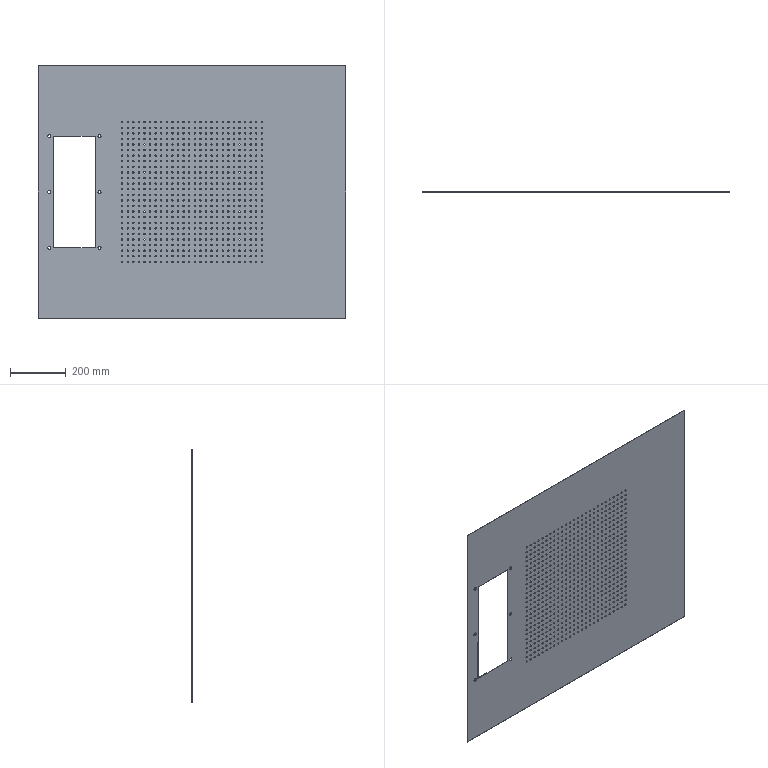Component | SolidWorks | BaseAssembly-1_BottomSealingPlate-1 | 1 solid | 1374 faces | volume 1841113 mm3 | cylinder 1364 | plane 10 | commonest cylinder face diameters 5 x1352 11 x12